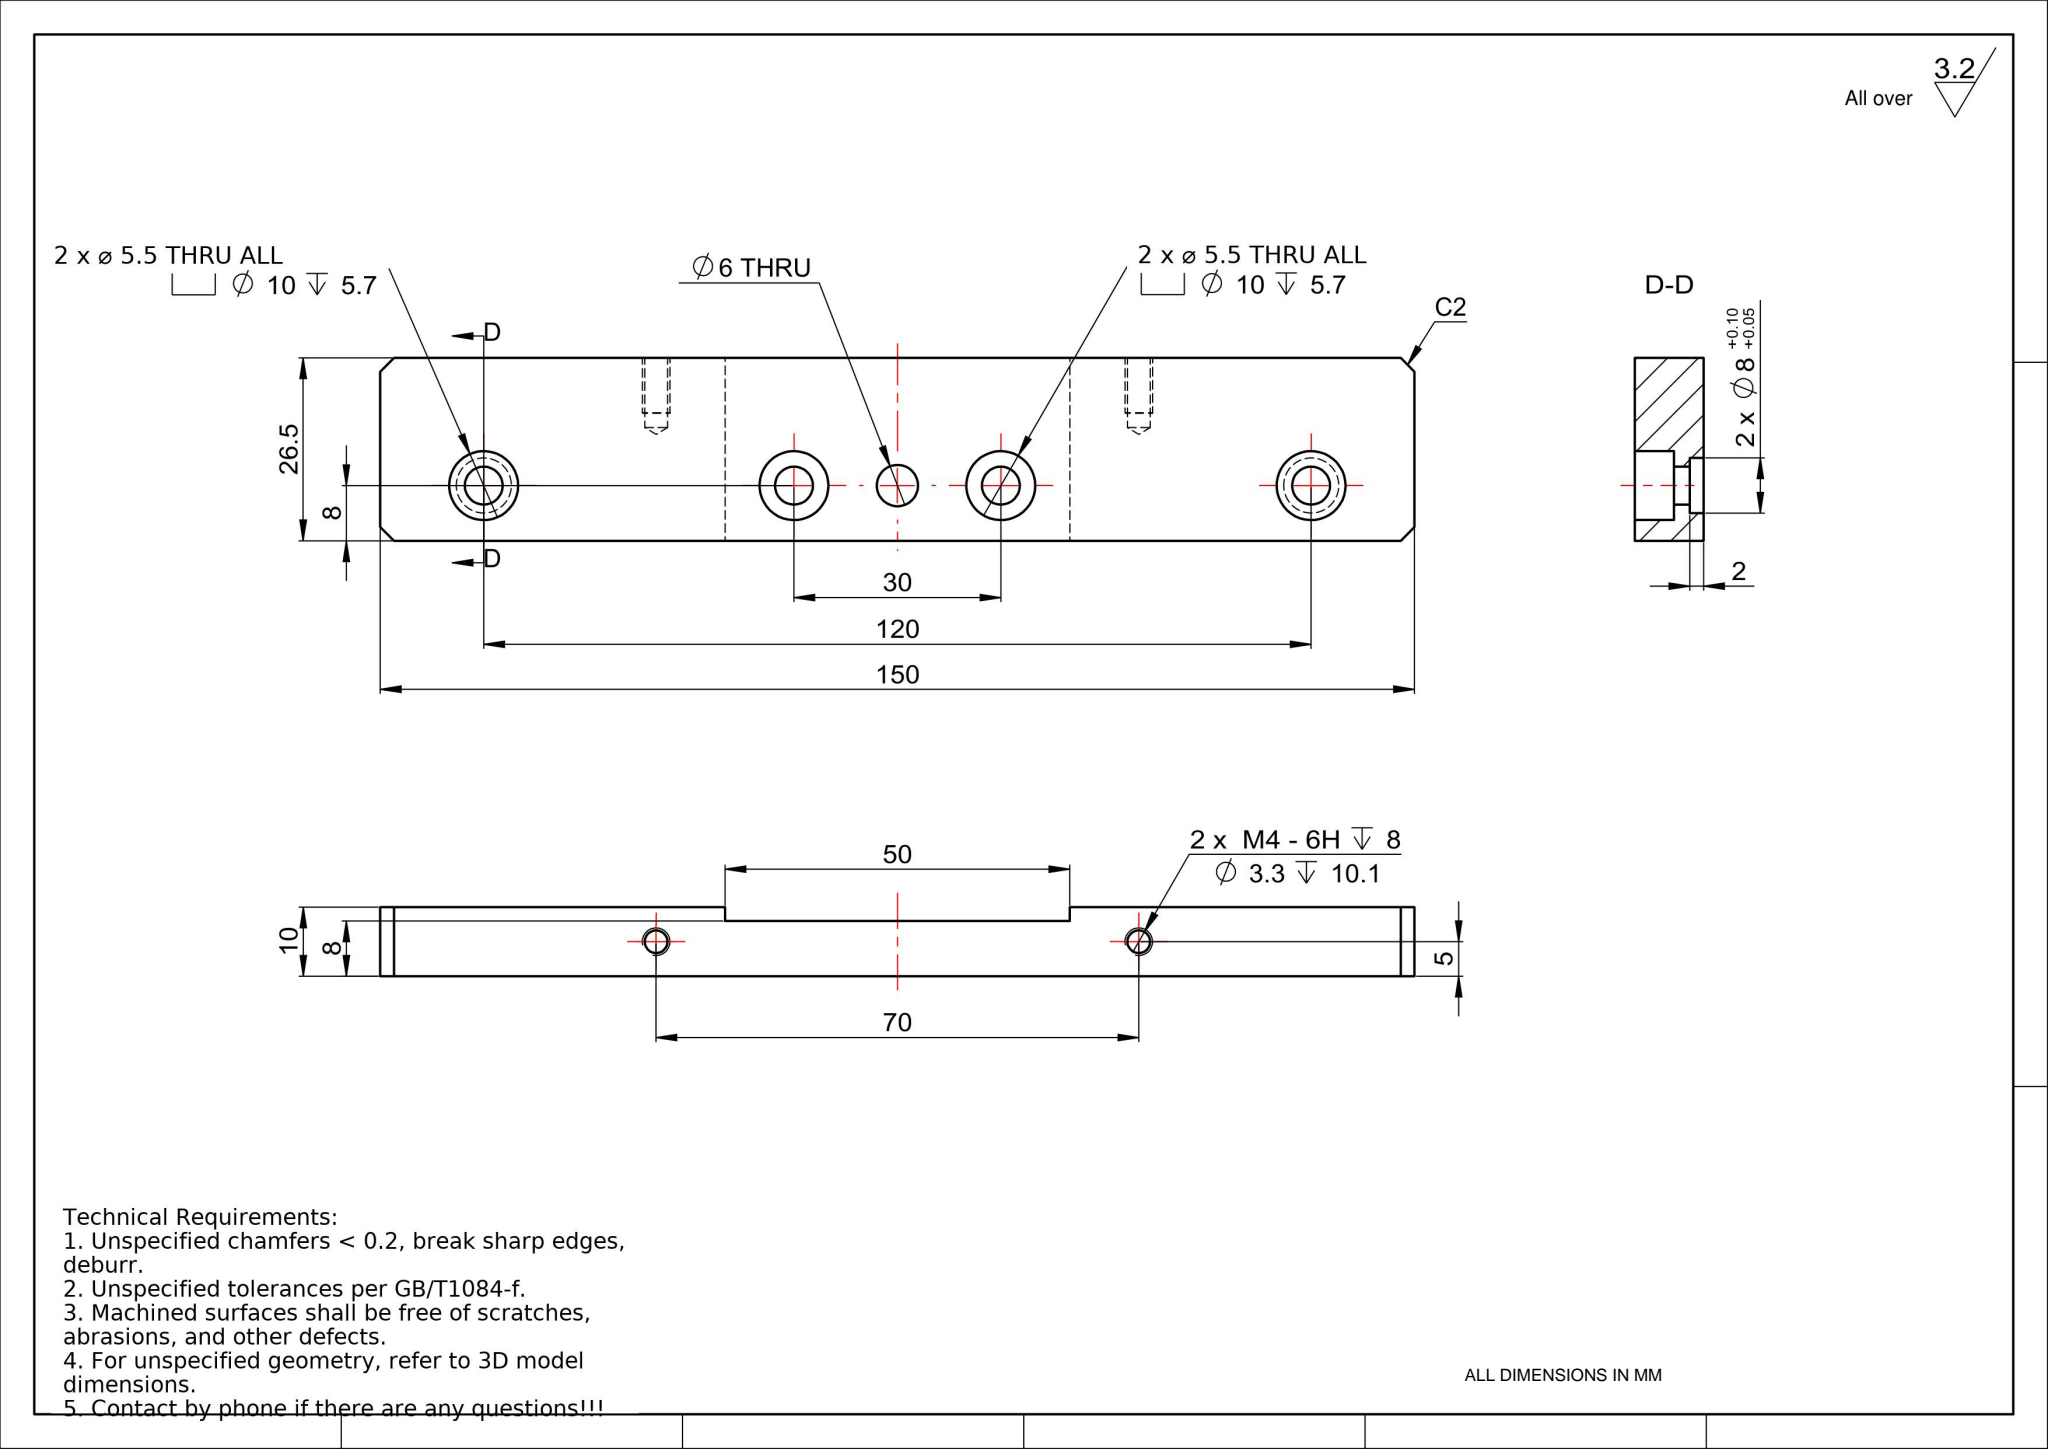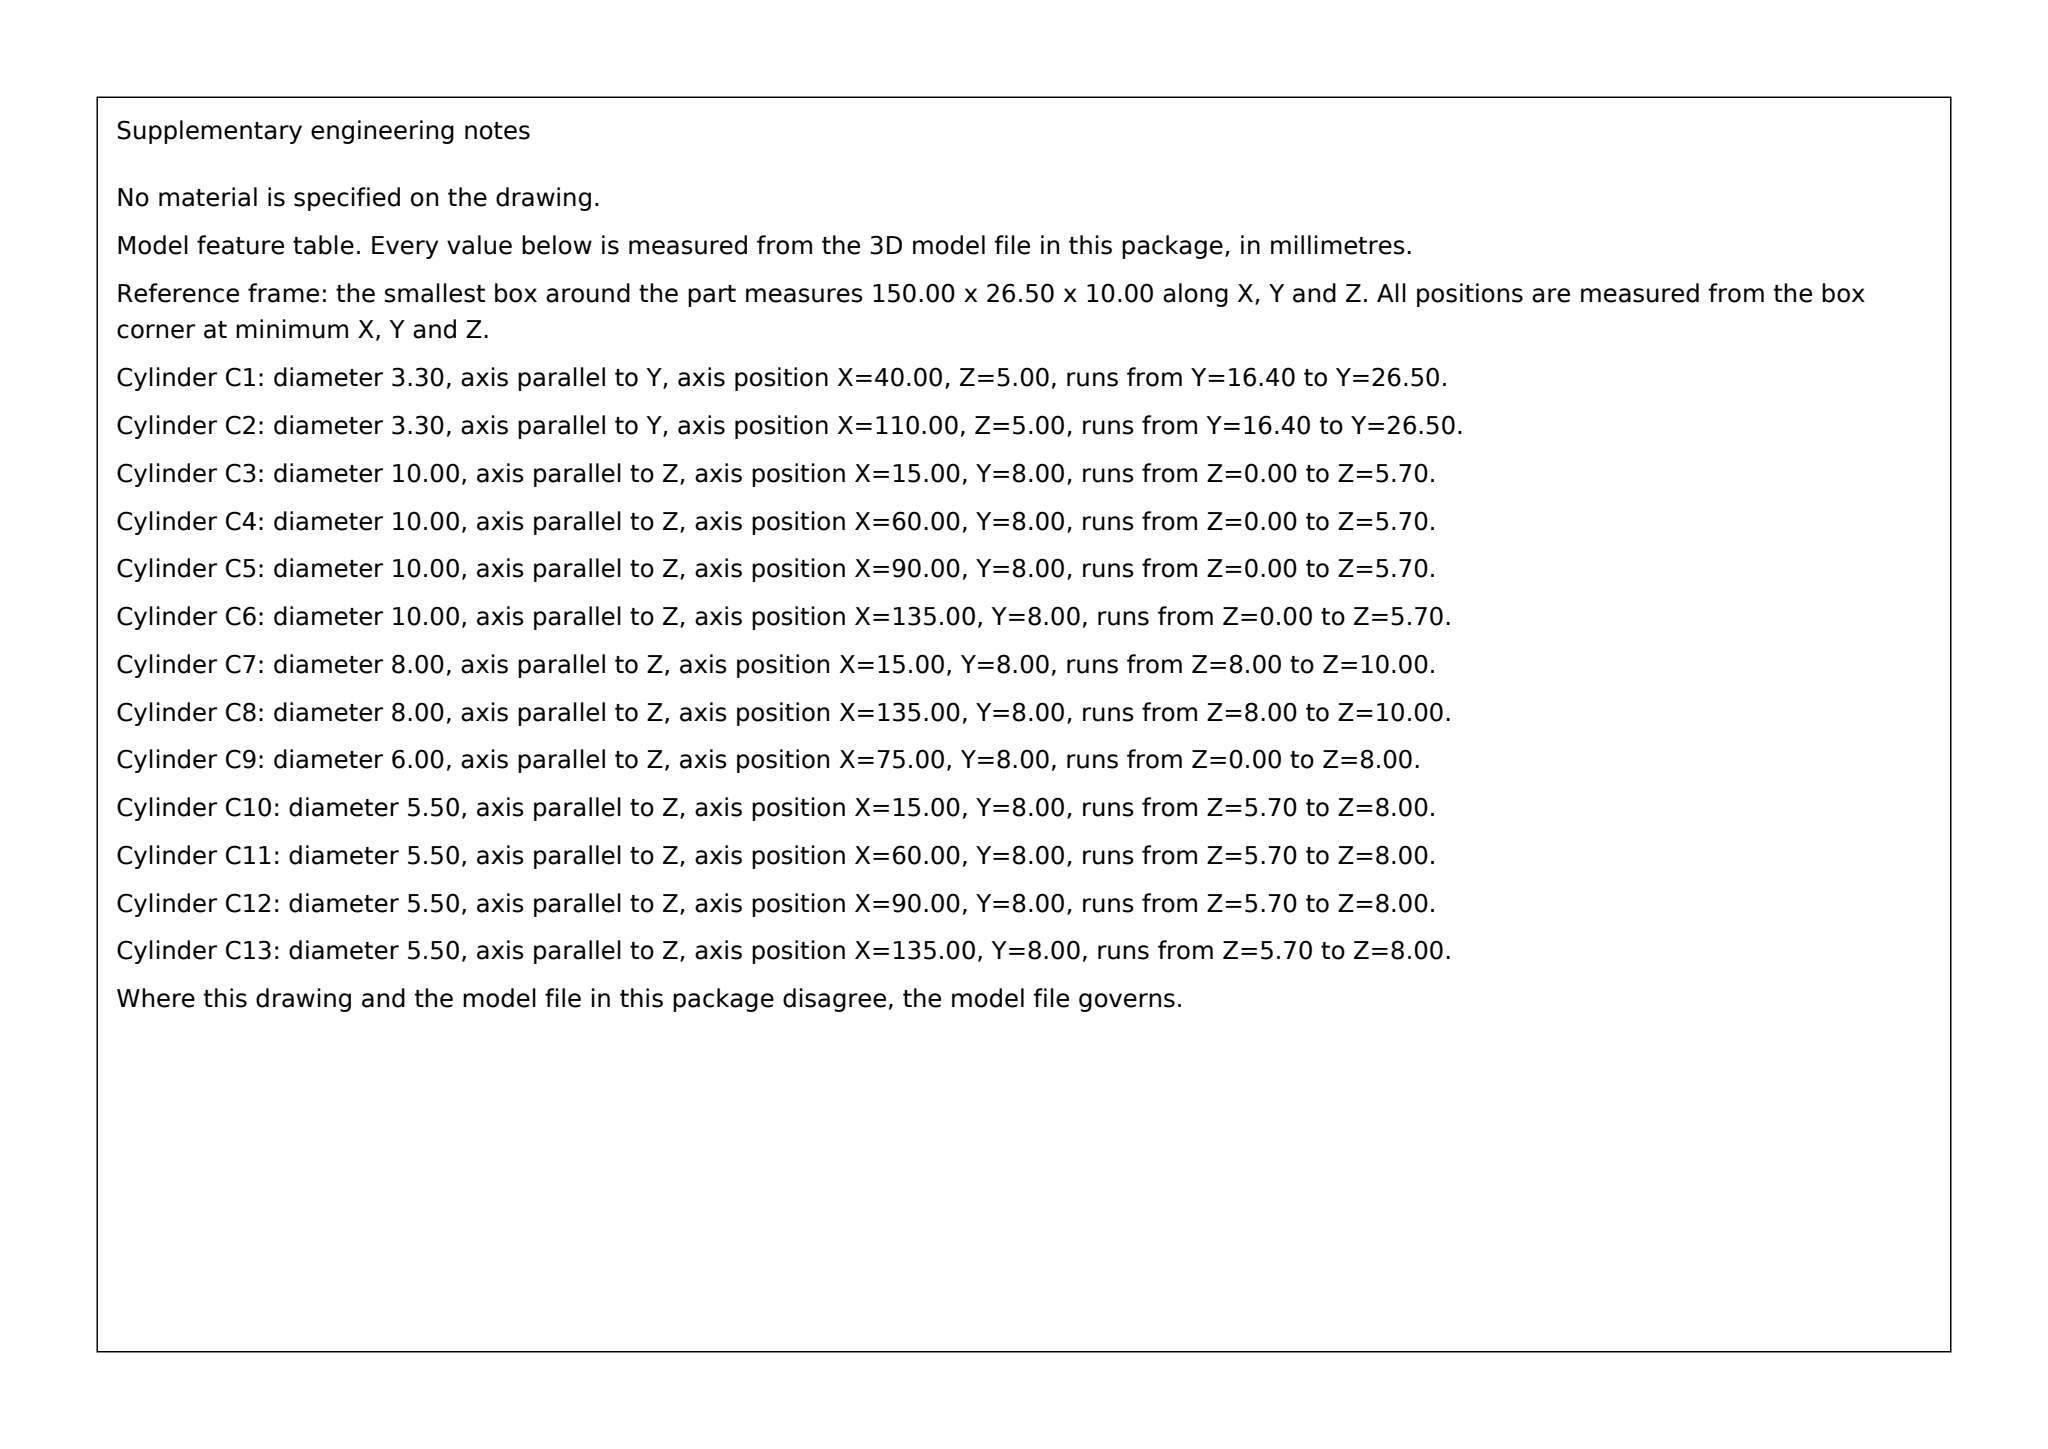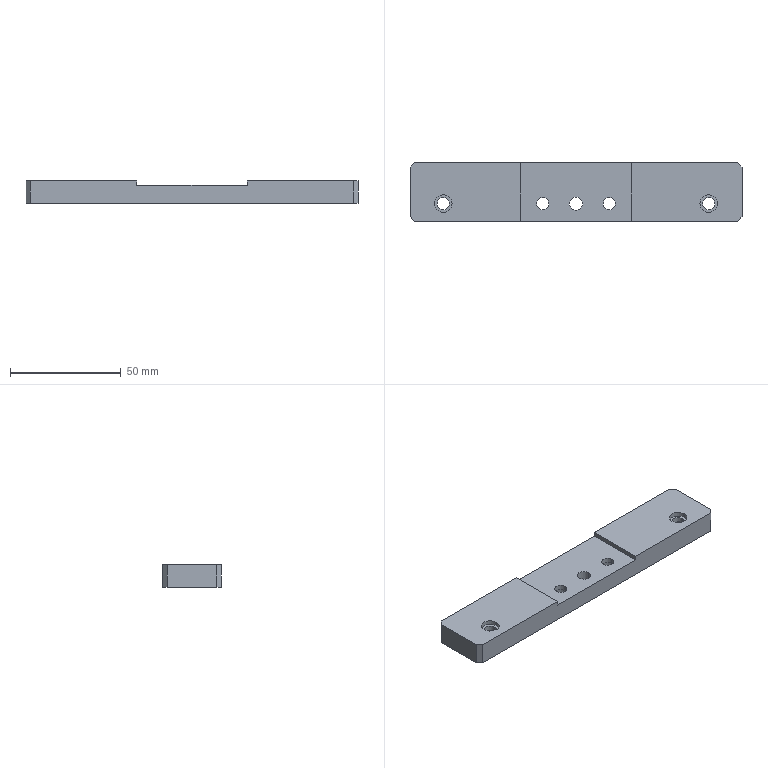Part | SolidWorks | mm | 1 solid | 50 faces | box 150 x 26.5 x 10 mm | volume 34405 mm3 | cylinder 26 | plane 20 | cone 4 | commonest cylinder face diameters 10 x8 5.5 x8 3.3 x4 8 x4 6 x2
build123d program:
from build123d import *

# Parameters (mm, degrees)
SKETCH1_W                                         = 180
SKETCH1_H                                         = 26.5
BOSS_EXTRUDE1_DEPTH                               = 5
SKETCH2_R                                         = 4
CUT_EXTRUDE1_DEPTH                                = 2
HOLE_SIZE_ACCORDING_TO_TYPE_1_OF_HEXA_D           = 5.5
HOLE_SIZE_ACCORDING_TO_TYPE_1_OF_HEXA_CBORE_D     = 10
HOLE_SIZE_ACCORDING_TO_TYPE_1_OF_HEXA_CBORE_DEPTH = 5.7
HOLE_SIZE_ACCORDING_TO_TYPE_2_OF_HEXA_D           = 5.5
HOLE_SIZE_ACCORDING_TO_TYPE_2_OF_HEXA_CBORE_D     = 10
HOLE_SIZE_ACCORDING_TO_TYPE_2_OF_HEXA_CBORE_DEPTH = 5.7
SKETCH12_W                                        = 50
SKETCH12_H                                        = 26.5
CUT_EXTRUDE4_DEPTH                                = 2
F_7_0_7_DIAMETER_HOLE1_D                          = 6
M4_TAPPED_HOLE1_D                                 = 3.3
M4_TAPPED_HOLE1_DEPTH                             = 10.1
M4_TAPPED_HOLE1_TIP                               = 0.9914
SKETCH18_W                                        = 15
SKETCH18_H                                        = 26.5
CUT_EXTRUDE5_DEPTH                                = 10
CHAMFER1_SIZE                                     = 2


with BuildPart() as part:
    # Sketch1 → Boss-Extrude1 (new, symmetric)
    with BuildSketch(Plane.XY):
        Rectangle(SKETCH1_W, SKETCH1_H)
    extrude(amount=BOSS_EXTRUDE1_DEPTH, both=True)

    # Sketch2 → Cut-Extrude1 (cut)
    with BuildSketch(Plane.XY.offset(5)):
        with Locations((-60, -5.25)):
            Circle(SKETCH2_R)
        with Locations((60, -5.25)):
            Circle(SKETCH2_R)
    extrude(amount=-CUT_EXTRUDE1_DEPTH, mode=Mode.SUBTRACT)

    # Hole Size _ according to_ type 1 of hexa (through all)
    with Locations(Plane(origin=(0, 0, -5), x_dir=(-1, 0, 0), z_dir=(0, 0, -1))):
        with Locations((-60, -5.25), (60, -5.25)):
            CounterBoreHole(HOLE_SIZE_ACCORDING_TO_TYPE_1_OF_HEXA_D / 2, HOLE_SIZE_ACCORDING_TO_TYPE_1_OF_HEXA_CBORE_D / 2, HOLE_SIZE_ACCORDING_TO_TYPE_1_OF_HEXA_CBORE_DEPTH)

    # Hole Size _ according to_ type 2 of hexa (through all)
    with Locations(Plane(origin=(0, 0, -5), x_dir=(-1, 0, 0), z_dir=(0, 0, -1))):
        with Locations((-15, -5.25), (15, -5.25)):
            CounterBoreHole(HOLE_SIZE_ACCORDING_TO_TYPE_2_OF_HEXA_D / 2, HOLE_SIZE_ACCORDING_TO_TYPE_2_OF_HEXA_CBORE_D / 2, HOLE_SIZE_ACCORDING_TO_TYPE_2_OF_HEXA_CBORE_DEPTH)

    # Sketch12 → Cut-Extrude4 (cut)
    with BuildSketch(Plane.XY.offset(5)):
        Rectangle(SKETCH12_W, SKETCH12_H)
    extrude(amount=-CUT_EXTRUDE4_DEPTH, mode=Mode.SUBTRACT)

    # 7.0 _7_ Diameter Hole1 (through all)
    with Locations(Plane(origin=(0, 0, -5), x_dir=(-1, 0, 0), z_dir=(0, 0, -1))):
        with Locations((0, -5.25)):
            Hole(F_7_0_7_DIAMETER_HOLE1_D / 2)

    # M4 Tapped Hole1
    with Locations(Plane(origin=(0, 13.25, 0), x_dir=(1, 0, 0), z_dir=(0, 1, 0))):
        with Locations((-35, 0), (35, 0)):
            Hole(M4_TAPPED_HOLE1_D / 2, depth=M4_TAPPED_HOLE1_DEPTH)
            with Locations((0, 0, -(M4_TAPPED_HOLE1_DEPTH + M4_TAPPED_HOLE1_TIP / 2))):  # 118° drill point
                Cone(0, M4_TAPPED_HOLE1_D / 2, M4_TAPPED_HOLE1_TIP, mode=Mode.SUBTRACT)

    # Sketch18 → Cut-Extrude5 (cut)
    with BuildSketch(Plane(origin=(0, 0, -5), x_dir=(-1, 0, 0), z_dir=(0, 0, -1))):
        with Locations((-82.5, 0)):
            Rectangle(SKETCH18_W, SKETCH18_H)
        with Locations((82.5, 0)):
            Rectangle(SKETCH18_W, SKETCH18_H)
    extrude(amount=-CUT_EXTRUDE5_DEPTH, mode=Mode.SUBTRACT)

    # Chamfer1
    chamfer1_edges = [part.edges().sort_by_distance(p)[0] for p in [
        (-75, -13.25, 0),
        (-75, 13.25, 0),
        (75, 13.25, 0),
        (75, -13.25, 0),
    ]]
    chamfer(chamfer1_edges, length=CHAMFER1_SIZE)


solid = part.part